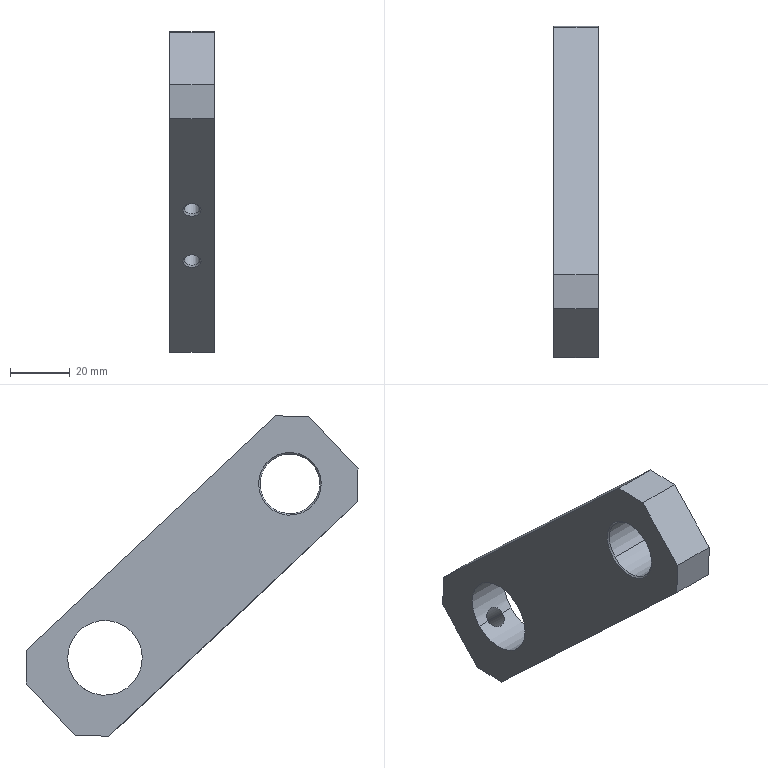Component | SolidWorks | FilmMechanism-3-1_LeftSupportBlock-1 | 1 solid | 32 faces | box 15 x 111.11 x 107.26 mm | volume 62724 mm3 | cone 12 | cylinder 10 | plane 10 | commonest cylinder face diameters 5 x4 6.8 x2 25 x2 20 x2
STEP:
#1=COLOUR_RGB('',0.7922,0.8196,0.9333);
#2=FILL_AREA_STYLE_COLOUR('',#1);
#3=FILL_AREA_STYLE('',(#2));
#4=SURFACE_STYLE_FILL_AREA(#3);
#5=SURFACE_SIDE_STYLE('',(#4));
#6=SURFACE_STYLE_USAGE(.BOTH.,#5);
#7=PRESENTATION_STYLE_ASSIGNMENT((#6));
#8=CARTESIAN_POINT('',(-21.419,17.638,-2.001));
#9=VERTEX_POINT('',#8);
#10=CARTESIAN_POINT('',(-21.222,17.638,-2.001));
#11=VERTEX_POINT('',#10);
#12=CARTESIAN_POINT('',(-21.321,17.638,-2.001));
#13=DIRECTION('',(0.,-0.6854,-0.7282));
#14=DIRECTION('',(1.,0.,0.));
#15=AXIS2_PLACEMENT_3D('',#12,#13,#14);
#16=CIRCLE('',#15,0.09843);
#17=EDGE_CURVE('',#9,#11,#16,.T.);
#18=ORIENTED_EDGE('',*,*,#17,.F.);
#19=CARTESIAN_POINT('',(-21.44,17.624,-2.016));
#20=VERTEX_POINT('',#19);
#21=CARTESIAN_POINT('',(-21.44,17.624,-2.016));
#22=DIRECTION('',(-0.7071,-0.4846,-0.5149));
#23=VECTOR('',#22,39.37);
#24=LINE('',#21,#23);
#25=EDGE_CURVE('',#9,#20,#24,.T.);
#26=ORIENTED_EDGE('',*,*,#25,.T.);
#27=CARTESIAN_POINT('',(-21.202,17.624,-2.016));
#28=VERTEX_POINT('',#27);
#29=CARTESIAN_POINT('',(-21.321,17.624,-2.016));
#30=DIRECTION('',(0.,-0.6854,-0.7282));
#31=DIRECTION('',(1.,0.,0.));
#32=AXIS2_PLACEMENT_3D('',#29,#30,#31);
#33=CIRCLE('',#32,0.1191);
#34=EDGE_CURVE('',#20,#28,#33,.T.);
#35=ORIENTED_EDGE('',*,*,#34,.T.);
#36=CARTESIAN_POINT('',(-21.202,17.624,-2.016));
#37=DIRECTION('',(0.7071,-0.4846,-0.5149));
#38=VECTOR('',#37,39.37);
#39=LINE('',#36,#38);
#40=EDGE_CURVE('',#11,#28,#39,.T.);
#41=ORIENTED_EDGE('',*,*,#40,.F.);
#42=EDGE_LOOP('',(#18,#26,#35,#41));
#43=FACE_OUTER_BOUND('',#42,.T.);
#44=CARTESIAN_POINT('',(-21.321,17.624,-2.016));
#45=DIRECTION('',(0.,-0.6854,-0.7282));
#46=DIRECTION('',(1.,0.,0.));
#47=AXIS2_PLACEMENT_3D('',#44,#45,#46);
#48=CONICAL_SURFACE('',#47,0.1191,0.7854);
#49=ADVANCED_FACE('',(#43),#48,.F.);
#50=CARTESIAN_POINT('',(-21.419,18.163,-1.443));
#51=VERTEX_POINT('',#50);
#52=CARTESIAN_POINT('',(-21.222,18.163,-1.443));
#53=VERTEX_POINT('',#52);
#54=CARTESIAN_POINT('',(-21.321,18.163,-1.443));
#55=DIRECTION('',(0.,-0.6854,-0.7282));
#56=DIRECTION('',(1.,0.,0.));
#57=AXIS2_PLACEMENT_3D('',#54,#55,#56);
#58=CIRCLE('',#57,0.09843);
#59=EDGE_CURVE('',#51,#53,#58,.T.);
#60=ORIENTED_EDGE('',*,*,#59,.F.);
#61=CARTESIAN_POINT('',(-21.419,17.624,-2.016));
#62=DIRECTION('',(0.,-0.6854,-0.7282));
#63=VECTOR('',#62,39.37);
#64=LINE('',#61,#63);
#65=EDGE_CURVE('',#51,#9,#64,.T.);
#66=ORIENTED_EDGE('',*,*,#65,.T.);
#67=ORIENTED_EDGE('',*,*,#17,.T.);
#68=CARTESIAN_POINT('',(-21.222,17.624,-2.016));
#69=DIRECTION('',(0.,-0.6854,-0.7282));
#70=VECTOR('',#69,39.37);
#71=LINE('',#68,#70);
#72=EDGE_CURVE('',#53,#11,#71,.T.);
#73=ORIENTED_EDGE('',*,*,#72,.F.);
#74=EDGE_LOOP('',(#60,#66,#67,#73));
#75=FACE_OUTER_BOUND('',#74,.T.);
#76=CARTESIAN_POINT('',(-21.321,17.624,-2.016));
#77=DIRECTION('',(0.,-0.6854,-0.7282));
#78=DIRECTION('',(1.,0.,0.));
#79=AXIS2_PLACEMENT_3D('',#76,#77,#78);
#80=CYLINDRICAL_SURFACE('',#79,0.09843);
#81=ADVANCED_FACE('',(#75),#80,.F.);
#82=CARTESIAN_POINT('',(-21.321,18.204,-1.4));
#83=VERTEX_POINT('',#82);
#84=CARTESIAN_POINT('',(-21.222,18.163,-1.443));
#85=DIRECTION('',(0.8572,-0.353,-0.375));
#86=VECTOR('',#85,39.37);
#87=LINE('',#84,#86);
#88=EDGE_CURVE('',#83,#53,#87,.T.);
#89=ORIENTED_EDGE('',*,*,#88,.F.);
#90=CARTESIAN_POINT('',(-21.419,18.163,-1.443));
#91=DIRECTION('',(-0.8572,-0.353,-0.375));
#92=VECTOR('',#91,39.37);
#93=LINE('',#90,#92);
#94=EDGE_CURVE('',#83,#51,#93,.T.);
#95=ORIENTED_EDGE('',*,*,#94,.T.);
#96=ORIENTED_EDGE('',*,*,#59,.T.);
#97=EDGE_LOOP('',(#89,#95,#96));
#98=FACE_OUTER_BOUND('',#97,.T.);
#99=CARTESIAN_POINT('',(-21.321,18.163,-1.443));
#100=DIRECTION('',(0.,-0.6854,-0.7282));
#101=DIRECTION('',(1.,0.,0.));
#102=AXIS2_PLACEMENT_3D('',#99,#100,#101);
#103=CONICAL_SURFACE('',#102,0.09843,1.03);
#104=ADVANCED_FACE('',(#98),#103,.F.);
#105=CARTESIAN_POINT('',(-21.419,16.921,-1.327));
#106=VERTEX_POINT('',#105);
#107=CARTESIAN_POINT('',(-21.222,16.921,-1.327));
#108=VERTEX_POINT('',#107);
#109=CARTESIAN_POINT('',(-21.321,16.921,-1.327));
#110=DIRECTION('',(0.,-0.6854,-0.7282));
#111=DIRECTION('',(1.,0.,0.));
#112=AXIS2_PLACEMENT_3D('',#109,#110,#111);
#113=CIRCLE('',#112,0.09843);
#114=EDGE_CURVE('',#106,#108,#113,.T.);
#115=ORIENTED_EDGE('',*,*,#114,.F.);
#116=CARTESIAN_POINT('',(-21.44,16.907,-1.342));
#117=VERTEX_POINT('',#116);
#118=CARTESIAN_POINT('',(-21.44,16.907,-1.342));
#119=DIRECTION('',(-0.7071,-0.4846,-0.5149));
#120=VECTOR('',#119,39.37);
#121=LINE('',#118,#120);
#122=EDGE_CURVE('',#106,#117,#121,.T.);
#123=ORIENTED_EDGE('',*,*,#122,.T.);
#124=CARTESIAN_POINT('',(-21.202,16.907,-1.342));
#125=VERTEX_POINT('',#124);
#126=CARTESIAN_POINT('',(-21.321,16.907,-1.342));
#127=DIRECTION('',(0.,-0.6854,-0.7282));
#128=DIRECTION('',(1.,0.,0.));
#129=AXIS2_PLACEMENT_3D('',#126,#127,#128);
#130=CIRCLE('',#129,0.1191);
#131=EDGE_CURVE('',#117,#125,#130,.T.);
#132=ORIENTED_EDGE('',*,*,#131,.T.);
#133=CARTESIAN_POINT('',(-21.202,16.907,-1.342));
#134=DIRECTION('',(0.7071,-0.4846,-0.5149));
#135=VECTOR('',#134,39.37);
#136=LINE('',#133,#135);
#137=EDGE_CURVE('',#108,#125,#136,.T.);
#138=ORIENTED_EDGE('',*,*,#137,.F.);
#139=EDGE_LOOP('',(#115,#123,#132,#138));
#140=FACE_OUTER_BOUND('',#139,.T.);
#141=CARTESIAN_POINT('',(-21.321,16.907,-1.342));
#142=DIRECTION('',(0.,-0.6854,-0.7282));
#143=DIRECTION('',(1.,0.,0.));
#144=AXIS2_PLACEMENT_3D('',#141,#142,#143);
#145=CONICAL_SURFACE('',#144,0.1191,0.7854);
#146=ADVANCED_FACE('',(#140),#145,.F.);
#147=CARTESIAN_POINT('',(-21.419,17.447,-0.7684));
#148=VERTEX_POINT('',#147);
#149=CARTESIAN_POINT('',(-21.222,17.447,-0.7684));
#150=VERTEX_POINT('',#149);
#151=CARTESIAN_POINT('',(-21.321,17.447,-0.7684));
#152=DIRECTION('',(0.,-0.6854,-0.7282));
#153=DIRECTION('',(1.,0.,0.));
#154=AXIS2_PLACEMENT_3D('',#151,#152,#153);
#155=CIRCLE('',#154,0.09843);
#156=EDGE_CURVE('',#148,#150,#155,.T.);
#157=ORIENTED_EDGE('',*,*,#156,.F.);
#158=CARTESIAN_POINT('',(-21.419,16.907,-1.342));
#159=DIRECTION('',(0.,-0.6854,-0.7282));
#160=VECTOR('',#159,39.37);
#161=LINE('',#158,#160);
#162=EDGE_CURVE('',#148,#106,#161,.T.);
#163=ORIENTED_EDGE('',*,*,#162,.T.);
#164=ORIENTED_EDGE('',*,*,#114,.T.);
#165=CARTESIAN_POINT('',(-21.222,16.907,-1.342));
#166=DIRECTION('',(0.,-0.6854,-0.7282));
#167=VECTOR('',#166,39.37);
#168=LINE('',#165,#167);
#169=EDGE_CURVE('',#150,#108,#168,.T.);
#170=ORIENTED_EDGE('',*,*,#169,.F.);
#171=EDGE_LOOP('',(#157,#163,#164,#170));
#172=FACE_OUTER_BOUND('',#171,.T.);
#173=CARTESIAN_POINT('',(-21.321,16.907,-1.342));
#174=DIRECTION('',(0.,-0.6854,-0.7282));
#175=DIRECTION('',(1.,0.,0.));
#176=AXIS2_PLACEMENT_3D('',#173,#174,#175);
#177=CYLINDRICAL_SURFACE('',#176,0.09843);
#178=ADVANCED_FACE('',(#172),#177,.F.);
#179=CARTESIAN_POINT('',(-21.321,17.487,-0.7253));
#180=VERTEX_POINT('',#179);
#181=CARTESIAN_POINT('',(-21.222,17.447,-0.7684));
#182=DIRECTION('',(0.8572,-0.353,-0.375));
#183=VECTOR('',#182,39.37);
#184=LINE('',#181,#183);
#185=EDGE_CURVE('',#180,#150,#184,.T.);
#186=ORIENTED_EDGE('',*,*,#185,.F.);
#187=CARTESIAN_POINT('',(-21.419,17.447,-0.7684));
#188=DIRECTION('',(-0.8572,-0.353,-0.375));
#189=VECTOR('',#188,39.37);
#190=LINE('',#187,#189);
#191=EDGE_CURVE('',#180,#148,#190,.T.);
#192=ORIENTED_EDGE('',*,*,#191,.T.);
#193=ORIENTED_EDGE('',*,*,#156,.T.);
#194=EDGE_LOOP('',(#186,#192,#193));
#195=FACE_OUTER_BOUND('',#194,.T.);
#196=CARTESIAN_POINT('',(-21.321,17.447,-0.7684));
#197=DIRECTION('',(0.,-0.6854,-0.7282));
#198=DIRECTION('',(1.,0.,0.));
#199=AXIS2_PLACEMENT_3D('',#196,#197,#198);
#200=CONICAL_SURFACE('',#199,0.09843,1.03);
#201=ADVANCED_FACE('',(#195),#200,.F.);
#202=CARTESIAN_POINT('',(-21.187,19.651,-2.843));
#203=VERTEX_POINT('',#202);
#204=CARTESIAN_POINT('',(-21.455,19.651,-2.843));
#205=VERTEX_POINT('',#204);
#206=CARTESIAN_POINT('',(-21.321,19.651,-2.843));
#207=DIRECTION('',(-0.,0.7282,-0.6854));
#208=DIRECTION('',(-1.,0.,0.));
#209=AXIS2_PLACEMENT_3D('',#206,#207,#208);
#210=CIRCLE('',#209,0.1339);
#211=EDGE_CURVE('',#203,#205,#210,.T.);
#212=ORIENTED_EDGE('',*,*,#211,.F.);
#213=CARTESIAN_POINT('',(-21.162,19.668,-2.86));
#214=VERTEX_POINT('',#213);
#215=CARTESIAN_POINT('',(-21.162,19.668,-2.86));
#216=DIRECTION('',(0.7071,0.5149,-0.4846));
#217=VECTOR('',#216,39.37);
#218=LINE('',#215,#217);
#219=EDGE_CURVE('',#203,#214,#218,.T.);
#220=ORIENTED_EDGE('',*,*,#219,.T.);
#221=CARTESIAN_POINT('',(-21.479,19.668,-2.86));
#222=VERTEX_POINT('',#221);
#223=CARTESIAN_POINT('',(-21.321,19.668,-2.86));
#224=DIRECTION('',(-0.,0.7282,-0.6854));
#225=DIRECTION('',(-1.,0.,0.));
#226=AXIS2_PLACEMENT_3D('',#223,#224,#225);
#227=CIRCLE('',#226,0.1585);
#228=EDGE_CURVE('',#214,#222,#227,.T.);
#229=ORIENTED_EDGE('',*,*,#228,.T.);
#230=CARTESIAN_POINT('',(-21.479,19.668,-2.86));
#231=DIRECTION('',(-0.7071,0.5149,-0.4846));
#232=VECTOR('',#231,39.37);
#233=LINE('',#230,#232);
#234=EDGE_CURVE('',#205,#222,#233,.T.);
#235=ORIENTED_EDGE('',*,*,#234,.F.);
#236=EDGE_LOOP('',(#212,#220,#229,#235));
#237=FACE_OUTER_BOUND('',#236,.T.);
#238=CARTESIAN_POINT('',(-21.321,19.668,-2.86));
#239=DIRECTION('',(-0.,0.7282,-0.6854));
#240=DIRECTION('',(-1.,0.,0.));
#241=AXIS2_PLACEMENT_3D('',#238,#239,#240);
#242=CONICAL_SURFACE('',#241,0.1585,0.7854);
#243=ADVANCED_FACE('',(#237),#242,.F.);
#244=CARTESIAN_POINT('',(-21.187,19.31,-2.522));
#245=VERTEX_POINT('',#244);
#246=CARTESIAN_POINT('',(-21.455,19.31,-2.522));
#247=VERTEX_POINT('',#246);
#248=CARTESIAN_POINT('',(-21.187,19.31,-2.522));
#249=CARTESIAN_POINT('',(-21.187,19.304,-2.529));
#250=CARTESIAN_POINT('',(-21.188,19.298,-2.535));
#251=CARTESIAN_POINT('',(-21.191,19.285,-2.547));
#252=CARTESIAN_POINT('',(-21.194,19.279,-2.553));
#253=CARTESIAN_POINT('',(-21.2,19.267,-2.563));
#254=CARTESIAN_POINT('',(-21.205,19.261,-2.568));
#255=CARTESIAN_POINT('',(-21.214,19.249,-2.577));
#256=CARTESIAN_POINT('',(-21.22,19.244,-2.581));
#257=CARTESIAN_POINT('',(-21.232,19.233,-2.589));
#258=CARTESIAN_POINT('',(-21.239,19.229,-2.592));
#259=CARTESIAN_POINT('',(-21.253,19.22,-2.597));
#260=CARTESIAN_POINT('',(-21.261,19.217,-2.6));
#261=CARTESIAN_POINT('',(-21.277,19.211,-2.603));
#262=CARTESIAN_POINT('',(-21.286,19.209,-2.605));
#263=CARTESIAN_POINT('',(-21.303,19.206,-2.607));
#264=CARTESIAN_POINT('',(-21.312,19.205,-2.607));
#265=CARTESIAN_POINT('',(-21.33,19.205,-2.607));
#266=CARTESIAN_POINT('',(-21.338,19.206,-2.607));
#267=CARTESIAN_POINT('',(-21.355,19.209,-2.605));
#268=CARTESIAN_POINT('',(-21.364,19.211,-2.603));
#269=CARTESIAN_POINT('',(-21.38,19.217,-2.6));
#270=CARTESIAN_POINT('',(-21.388,19.22,-2.597));
#271=CARTESIAN_POINT('',(-21.402,19.229,-2.592));
#272=CARTESIAN_POINT('',(-21.409,19.233,-2.589));
#273=CARTESIAN_POINT('',(-21.421,19.244,-2.581));
#274=CARTESIAN_POINT('',(-21.427,19.249,-2.577));
#275=CARTESIAN_POINT('',(-21.437,19.261,-2.568));
#276=CARTESIAN_POINT('',(-21.441,19.267,-2.563));
#277=CARTESIAN_POINT('',(-21.448,19.279,-2.553));
#278=CARTESIAN_POINT('',(-21.45,19.285,-2.547));
#279=CARTESIAN_POINT('',(-21.454,19.298,-2.535));
#280=CARTESIAN_POINT('',(-21.455,19.304,-2.529));
#281=CARTESIAN_POINT('',(-21.455,19.31,-2.522));
#282=B_SPLINE_CURVE_WITH_KNOTS('',3,(#248,#249,#250,#251,#252,#253,#254,#255,#256,#257,#258,#259,#260,#261,#262,#263,#264,#265,#266,#267,#268,#269,#270,#271,#272,#273,#274,#275,#276,#277,#278,#279,#280,#281),.UNSPECIFIED.,.F.,.F.,(4,2,2,2,2,2,2,2,2,2,2,2,2,2,2,2,4),(0.01068,0.01135,0.01202,0.01268,0.01335,0.01402,0.01468,0.01535,0.01602,0.01669,0.01735,0.01802,0.01869,0.01936,0.02002,0.02069,0.02136),.UNSPECIFIED.);
#283=EDGE_CURVE('',#245,#247,#282,.T.);
#284=ORIENTED_EDGE('',*,*,#283,.F.);
#285=CARTESIAN_POINT('',(-21.187,19.668,-2.86));
#286=DIRECTION('',(-0.,0.7282,-0.6854));
#287=VECTOR('',#286,39.37);
#288=LINE('',#285,#287);
#289=EDGE_CURVE('',#245,#203,#288,.T.);
#290=ORIENTED_EDGE('',*,*,#289,.T.);
#291=ORIENTED_EDGE('',*,*,#211,.T.);
#292=CARTESIAN_POINT('',(-21.455,19.668,-2.86));
#293=DIRECTION('',(-0.,0.7282,-0.6854));
#294=VECTOR('',#293,39.37);
#295=LINE('',#292,#294);
#296=EDGE_CURVE('',#247,#205,#295,.T.);
#297=ORIENTED_EDGE('',*,*,#296,.F.);
#298=EDGE_LOOP('',(#284,#290,#291,#297));
#299=FACE_OUTER_BOUND('',#298,.T.);
#300=CARTESIAN_POINT('',(-21.321,19.668,-2.86));
#301=DIRECTION('',(-0.,0.7282,-0.6854));
#302=DIRECTION('',(-1.,0.,0.));
#303=AXIS2_PLACEMENT_3D('',#300,#301,#302);
#304=CYLINDRICAL_SURFACE('',#303,0.1339);
#305=ADVANCED_FACE('',(#299),#304,.F.);
#306=CARTESIAN_POINT('',(-21.616,18.593,-1.848));
#307=VERTEX_POINT('',#306);
#308=CARTESIAN_POINT('',(-21.616,19.31,-2.522));
#309=VERTEX_POINT('',#308);
#310=CARTESIAN_POINT('',(-21.616,18.952,-2.185));
#311=DIRECTION('',(1.,0.,0.));
#312=DIRECTION('',(0.,0.7282,-0.6854));
#313=AXIS2_PLACEMENT_3D('',#310,#311,#312);
#314=CIRCLE('',#313,0.4921);
#315=EDGE_CURVE('',#307,#309,#314,.T.);
#316=ORIENTED_EDGE('',*,*,#315,.F.);
#317=CARTESIAN_POINT('',(-21.025,18.593,-1.848));
#318=VERTEX_POINT('',#317);
#319=CARTESIAN_POINT('',(-21.025,18.593,-1.848));
#320=DIRECTION('',(1.,0.,0.));
#321=VECTOR('',#320,39.37);
#322=LINE('',#319,#321);
#323=EDGE_CURVE('',#307,#318,#322,.T.);
#324=ORIENTED_EDGE('',*,*,#323,.T.);
#325=CARTESIAN_POINT('',(-21.025,19.31,-2.522));
#326=VERTEX_POINT('',#325);
#327=CARTESIAN_POINT('',(-21.025,18.952,-2.185));
#328=DIRECTION('',(1.,0.,0.));
#329=DIRECTION('',(0.,0.7282,-0.6854));
#330=AXIS2_PLACEMENT_3D('',#327,#328,#329);
#331=CIRCLE('',#330,0.4921);
#332=EDGE_CURVE('',#318,#326,#331,.T.);
#333=ORIENTED_EDGE('',*,*,#332,.T.);
#334=CARTESIAN_POINT('',(-21.025,19.31,-2.522));
#335=DIRECTION('',(1.,0.,0.));
#336=VECTOR('',#335,39.37);
#337=LINE('',#334,#336);
#338=EDGE_CURVE('',#245,#326,#337,.T.);
#339=ORIENTED_EDGE('',*,*,#338,.F.);
#340=ORIENTED_EDGE('',*,*,#283,.T.);
#341=CARTESIAN_POINT('',(-21.025,19.31,-2.522));
#342=DIRECTION('',(1.,0.,0.));
#343=VECTOR('',#342,39.37);
#344=LINE('',#341,#343);
#345=EDGE_CURVE('',#309,#247,#344,.T.);
#346=ORIENTED_EDGE('',*,*,#345,.F.);
#347=EDGE_LOOP('',(#316,#324,#333,#339,#340,#346));
#348=FACE_OUTER_BOUND('',#347,.T.);
#349=CARTESIAN_POINT('',(-21.025,18.952,-2.185));
#350=DIRECTION('',(1.,0.,0.));
#351=DIRECTION('',(0.,0.7282,-0.6854));
#352=AXIS2_PLACEMENT_3D('',#349,#350,#351);
#353=CYLINDRICAL_SURFACE('',#352,0.4921);
#354=ADVANCED_FACE('',(#348),#353,.F.);
#355=CARTESIAN_POINT('',(-21.596,16.802,-0.1613));
#356=VERTEX_POINT('',#355);
#357=CARTESIAN_POINT('',(-21.596,16.228,0.3784));
#358=VERTEX_POINT('',#357);
#359=CARTESIAN_POINT('',(-21.596,16.515,0.1086));
#360=DIRECTION('',(-1.,-0.,-0.));
#361=DIRECTION('',(0.,-0.7282,0.6854));
#362=AXIS2_PLACEMENT_3D('',#359,#360,#361);
#363=CIRCLE('',#362,0.3937);
#364=EDGE_CURVE('',#356,#358,#363,.T.);
#365=ORIENTED_EDGE('',*,*,#364,.F.);
#366=CARTESIAN_POINT('',(-21.616,16.816,-0.1748));
#367=VERTEX_POINT('',#366);
#368=CARTESIAN_POINT('',(-21.616,16.816,-0.1748));
#369=DIRECTION('',(-0.7071,0.5149,-0.4846));
#370=VECTOR('',#369,39.37);
#371=LINE('',#368,#370);
#372=EDGE_CURVE('',#356,#367,#371,.T.);
#373=ORIENTED_EDGE('',*,*,#372,.T.);
#374=CARTESIAN_POINT('',(-21.616,16.214,0.3919));
#375=VERTEX_POINT('',#374);
#376=CARTESIAN_POINT('',(-21.616,16.515,0.1086));
#377=DIRECTION('',(-1.,-0.,-0.));
#378=DIRECTION('',(0.,-0.7282,0.6854));
#379=AXIS2_PLACEMENT_3D('',#376,#377,#378);
#380=CIRCLE('',#379,0.4134);
#381=EDGE_CURVE('',#367,#375,#380,.T.);
#382=ORIENTED_EDGE('',*,*,#381,.T.);
#383=CARTESIAN_POINT('',(-21.616,16.214,0.3919));
#384=DIRECTION('',(-0.7071,-0.5149,0.4846));
#385=VECTOR('',#384,39.37);
#386=LINE('',#383,#385);
#387=EDGE_CURVE('',#358,#375,#386,.T.);
#388=ORIENTED_EDGE('',*,*,#387,.F.);
#389=EDGE_LOOP('',(#365,#373,#382,#388));
#390=FACE_OUTER_BOUND('',#389,.T.);
#391=CARTESIAN_POINT('',(-21.616,16.515,0.1086));
#392=DIRECTION('',(-1.,-0.,-0.));
#393=DIRECTION('',(0.,-0.7282,0.6854));
#394=AXIS2_PLACEMENT_3D('',#391,#392,#393);
#395=CONICAL_SURFACE('',#394,0.4134,0.7854);
#396=ADVANCED_FACE('',(#390),#395,.F.);
#397=CARTESIAN_POINT('',(-21.025,16.802,-0.1613));
#398=VERTEX_POINT('',#397);
#399=CARTESIAN_POINT('',(-21.025,16.228,0.3784));
#400=VERTEX_POINT('',#399);
#401=CARTESIAN_POINT('',(-21.025,16.515,0.1086));
#402=DIRECTION('',(-1.,-0.,-0.));
#403=DIRECTION('',(0.,-0.7282,0.6854));
#404=AXIS2_PLACEMENT_3D('',#401,#402,#403);
#405=CIRCLE('',#404,0.3937);
#406=EDGE_CURVE('',#398,#400,#405,.T.);
#407=ORIENTED_EDGE('',*,*,#406,.F.);
#408=CARTESIAN_POINT('',(-21.616,16.802,-0.1613));
#409=DIRECTION('',(-1.,-0.,-0.));
#410=VECTOR('',#409,39.37);
#411=LINE('',#408,#410);
#412=EDGE_CURVE('',#398,#356,#411,.T.);
#413=ORIENTED_EDGE('',*,*,#412,.T.);
#414=ORIENTED_EDGE('',*,*,#364,.T.);
#415=CARTESIAN_POINT('',(-21.616,16.228,0.3784));
#416=DIRECTION('',(-1.,-0.,-0.));
#417=VECTOR('',#416,39.37);
#418=LINE('',#415,#417);
#419=EDGE_CURVE('',#400,#358,#418,.T.);
#420=ORIENTED_EDGE('',*,*,#419,.F.);
#421=EDGE_LOOP('',(#407,#413,#414,#420));
#422=FACE_OUTER_BOUND('',#421,.T.);
#423=CARTESIAN_POINT('',(-21.616,16.515,0.1086));
#424=DIRECTION('',(-1.,-0.,-0.));
#425=DIRECTION('',(0.,-0.7282,0.6854));
#426=AXIS2_PLACEMENT_3D('',#423,#424,#425);
#427=CYLINDRICAL_SURFACE('',#426,0.3937);
#428=ADVANCED_FACE('',(#422),#427,.F.);
#429=CARTESIAN_POINT('',(-21.616,19.979,-2.07));
#430=VERTEX_POINT('',#429);
#431=CARTESIAN_POINT('',(-21.616,19.992,-2.516));
#432=VERTEX_POINT('',#431);
#433=CARTESIAN_POINT('',(-21.616,19.979,-2.07));
#434=DIRECTION('',(-0.,0.03026,-0.9995));
#435=VECTOR('',#434,39.37);
#436=LINE('',#433,#435);
#437=EDGE_CURVE('',#430,#432,#436,.T.);
#438=ORIENTED_EDGE('',*,*,#437,.F.);
#439=CARTESIAN_POINT('',(-21.025,19.979,-2.07));
#440=VERTEX_POINT('',#439);
#441=CARTESIAN_POINT('',(-21.025,19.979,-2.07));
#442=DIRECTION('',(-1.,-0.,-0.));
#443=VECTOR('',#442,39.37);
#444=LINE('',#441,#443);
#445=EDGE_CURVE('',#440,#430,#444,.T.);
#446=ORIENTED_EDGE('',*,*,#445,.F.);
#447=CARTESIAN_POINT('',(-21.025,19.992,-2.516));
#448=VERTEX_POINT('',#447);
#449=CARTESIAN_POINT('',(-21.025,19.979,-2.07));
#450=DIRECTION('',(-0.,0.03026,-0.9995));
#451=VECTOR('',#450,39.37);
#452=LINE('',#449,#451);
#453=EDGE_CURVE('',#440,#448,#452,.T.);
#454=ORIENTED_EDGE('',*,*,#453,.T.);
#455=CARTESIAN_POINT('',(-21.025,19.992,-2.516));
#456=DIRECTION('',(-1.,-0.,-0.));
#457=VECTOR('',#456,39.37);
#458=LINE('',#455,#457);
#459=EDGE_CURVE('',#448,#432,#458,.T.);
#460=ORIENTED_EDGE('',*,*,#459,.T.);
#461=EDGE_LOOP('',(#438,#446,#454,#460));
#462=FACE_OUTER_BOUND('',#461,.T.);
#463=CARTESIAN_POINT('',(-21.025,19.979,-2.07));
#464=DIRECTION('',(-0.,0.9995,0.03026));
#465=DIRECTION('',(-0.,0.03026,-0.9995));
#466=AXIS2_PLACEMENT_3D('',#463,#464,#465);
#467=PLANE('',#466);
#468=ADVANCED_FACE('',(#462),#467,.T.);
#469=CARTESIAN_POINT('',(-21.616,16.711,1.006));
#470=VERTEX_POINT('',#469);
#471=CARTESIAN_POINT('',(-21.616,16.711,1.006));
#472=DIRECTION('',(-0.,0.7282,-0.6854));
#473=VECTOR('',#472,39.37);
#474=LINE('',#471,#473);
#475=EDGE_CURVE('',#470,#430,#474,.T.);
#476=ORIENTED_EDGE('',*,*,#475,.F.);
#477=CARTESIAN_POINT('',(-21.025,16.711,1.006));
#478=VERTEX_POINT('',#477);
#479=CARTESIAN_POINT('',(-21.025,16.711,1.006));
#480=DIRECTION('',(-1.,-0.,-0.));
#481=VECTOR('',#480,39.37);
#482=LINE('',#479,#481);
#483=EDGE_CURVE('',#478,#470,#482,.T.);
#484=ORIENTED_EDGE('',*,*,#483,.F.);
#485=CARTESIAN_POINT('',(-21.025,16.711,1.006));
#486=DIRECTION('',(-0.,0.7282,-0.6854));
#487=VECTOR('',#486,39.37);
#488=LINE('',#485,#487);
#489=EDGE_CURVE('',#478,#440,#488,.T.);
#490=ORIENTED_EDGE('',*,*,#489,.T.);
#491=ORIENTED_EDGE('',*,*,#445,.T.);
#492=EDGE_LOOP('',(#476,#484,#490,#491));
#493=FACE_OUTER_BOUND('',#492,.T.);
#494=CARTESIAN_POINT('',(-21.025,16.711,1.006));
#495=DIRECTION('',(-0.,0.6854,0.7282));
#496=DIRECTION('',(-1.,-0.,-0.));
#497=AXIS2_PLACEMENT_3D('',#494,#495,#496);
#498=PLANE('',#497);
#499=ADVANCED_FACE('',(#493),#498,.T.);
#500=CARTESIAN_POINT('',(-21.616,16.265,0.9923));
#501=VERTEX_POINT('',#500);
#502=CARTESIAN_POINT('',(-21.616,16.265,0.9923));
#503=DIRECTION('',(-0.,0.9995,0.03026));
#504=VECTOR('',#503,39.37);
#505=LINE('',#502,#504);
#506=EDGE_CURVE('',#501,#470,#505,.T.);
#507=ORIENTED_EDGE('',*,*,#506,.F.);
#508=CARTESIAN_POINT('',(-21.025,16.265,0.9923));
#509=VERTEX_POINT('',#508);
#510=CARTESIAN_POINT('',(-21.025,16.265,0.9923));
#511=DIRECTION('',(-1.,-0.,-0.));
#512=VECTOR('',#511,39.37);
#513=LINE('',#510,#512);
#514=EDGE_CURVE('',#509,#501,#513,.T.);
#515=ORIENTED_EDGE('',*,*,#514,.F.);
#516=CARTESIAN_POINT('',(-21.025,16.265,0.9923));
#517=DIRECTION('',(-0.,0.9995,0.03026));
#518=VECTOR('',#517,39.37);
#519=LINE('',#516,#518);
#520=EDGE_CURVE('',#509,#478,#519,.T.);
#521=ORIENTED_EDGE('',*,*,#520,.T.);
#522=ORIENTED_EDGE('',*,*,#483,.T.);
#523=EDGE_LOOP('',(#507,#515,#521,#522));
#524=FACE_OUTER_BOUND('',#523,.T.);
#525=CARTESIAN_POINT('',(-21.025,16.265,0.9923));
#526=DIRECTION('',(0.,-0.03026,0.9995));
#527=DIRECTION('',(-0.,0.9995,0.03026));
#528=AXIS2_PLACEMENT_3D('',#525,#526,#527);
#529=PLANE('',#528);
#530=ADVANCED_FACE('',(#524),#529,.T.);
#531=CARTESIAN_POINT('',(-21.616,15.618,0.3042));
#532=VERTEX_POINT('',#531);
#533=CARTESIAN_POINT('',(-21.616,15.618,0.3042));
#534=DIRECTION('',(-0.,0.6854,0.7282));
#535=VECTOR('',#534,39.37);
#536=LINE('',#533,#535);
#537=EDGE_CURVE('',#532,#501,#536,.T.);
#538=ORIENTED_EDGE('',*,*,#537,.F.);
#539=CARTESIAN_POINT('',(-21.025,15.618,0.3042));
#540=VERTEX_POINT('',#539);
#541=CARTESIAN_POINT('',(-21.025,15.618,0.3042));
#542=DIRECTION('',(-1.,-0.,-0.));
#543=VECTOR('',#542,39.37);
#544=LINE('',#541,#543);
#545=EDGE_CURVE('',#540,#532,#544,.T.);
#546=ORIENTED_EDGE('',*,*,#545,.F.);
#547=CARTESIAN_POINT('',(-21.025,15.618,0.3042));
#548=DIRECTION('',(-0.,0.6854,0.7282));
#549=VECTOR('',#548,39.37);
#550=LINE('',#547,#549);
#551=EDGE_CURVE('',#540,#509,#550,.T.);
#552=ORIENTED_EDGE('',*,*,#551,.T.);
#553=ORIENTED_EDGE('',*,*,#514,.T.);
#554=EDGE_LOOP('',(#538,#546,#552,#553));
#555=FACE_OUTER_BOUND('',#554,.T.);
#556=CARTESIAN_POINT('',(-21.025,15.618,0.3042));
#557=DIRECTION('',(0.,-0.7282,0.6854));
#558=DIRECTION('',(1.,0.,0.));
#559=AXIS2_PLACEMENT_3D('',#556,#557,#558);
#560=PLANE('',#559);
#561=ADVANCED_FACE('',(#555),#560,.T.);
#562=CARTESIAN_POINT('',(-21.616,15.631,-0.141));
#563=VERTEX_POINT('',#562);
#564=CARTESIAN_POINT('',(-21.616,15.631,-0.141));
#565=DIRECTION('',(0.,-0.03026,0.9995));
#566=VECTOR('',#565,39.37);
#567=LINE('',#564,#566);
#568=EDGE_CURVE('',#563,#532,#567,.T.);
#569=ORIENTED_EDGE('',*,*,#568,.F.);
#570=CARTESIAN_POINT('',(-21.025,15.631,-0.141));
#571=VERTEX_POINT('',#570);
#572=CARTESIAN_POINT('',(-21.025,15.631,-0.141));
#573=DIRECTION('',(-1.,-0.,-0.));
#574=VECTOR('',#573,39.37);
#575=LINE('',#572,#574);
#576=EDGE_CURVE('',#571,#563,#575,.T.);
#577=ORIENTED_EDGE('',*,*,#576,.F.);
#578=CARTESIAN_POINT('',(-21.025,15.631,-0.141));
#579=DIRECTION('',(0.,-0.03026,0.9995));
#580=VECTOR('',#579,39.37);
#581=LINE('',#578,#580);
#582=EDGE_CURVE('',#571,#540,#581,.T.);
#583=ORIENTED_EDGE('',*,*,#582,.T.);
#584=ORIENTED_EDGE('',*,*,#545,.T.);
#585=EDGE_LOOP('',(#569,#577,#583,#584));
#586=FACE_OUTER_BOUND('',#585,.T.);
#587=CARTESIAN_POINT('',(-21.025,15.631,-0.141));
#588=DIRECTION('',(0.,-0.9995,-0.03026));
#589=DIRECTION('',(0.,-0.03026,0.9995));
#590=AXIS2_PLACEMENT_3D('',#587,#588,#589);
#591=PLANE('',#590);
#592=ADVANCED_FACE('',(#586),#591,.T.);
#593=CARTESIAN_POINT('',(-21.321,17.624,-2.016));
#594=DIRECTION('',(0.,-0.6854,-0.7282));
#595=DIRECTION('',(1.,0.,0.));
#596=AXIS2_PLACEMENT_3D('',#593,#594,#595);
#597=CIRCLE('',#596,0.1191);
#598=EDGE_CURVE('',#28,#20,#597,.T.);
#599=ORIENTED_EDGE('',*,*,#598,.F.);
#600=ORIENTED_EDGE('',*,*,#34,.F.);
#601=EDGE_LOOP('',(#599,#600));
#602=FACE_BOUND('',#601,.T.);
#603=CARTESIAN_POINT('',(-21.321,16.907,-1.342));
#604=DIRECTION('',(0.,-0.6854,-0.7282));
#605=DIRECTION('',(1.,0.,0.));
#606=AXIS2_PLACEMENT_3D('',#603,#604,#605);
#607=CIRCLE('',#606,0.1191);
#608=EDGE_CURVE('',#125,#117,#607,.T.);
#609=ORIENTED_EDGE('',*,*,#608,.F.);
#610=ORIENTED_EDGE('',*,*,#131,.F.);
#611=EDGE_LOOP('',(#609,#610));
#612=FACE_BOUND('',#611,.T.);
#613=CARTESIAN_POINT('',(-21.616,18.899,-3.217));
#614=VERTEX_POINT('',#613);
#615=CARTESIAN_POINT('',(-21.616,18.899,-3.217));
#616=DIRECTION('',(0.,-0.7282,0.6854));
#617=VECTOR('',#616,39.37);
#618=LINE('',#615,#617);
#619=EDGE_CURVE('',#614,#563,#618,.T.);
#620=ORIENTED_EDGE('',*,*,#619,.F.);
#621=CARTESIAN_POINT('',(-21.025,18.899,-3.217));
#622=VERTEX_POINT('',#621);
#623=CARTESIAN_POINT('',(-21.025,18.899,-3.217));
#624=DIRECTION('',(-1.,-0.,-0.));
#625=VECTOR('',#624,39.37);
#626=LINE('',#623,#625);
#627=EDGE_CURVE('',#622,#614,#626,.T.);
#628=ORIENTED_EDGE('',*,*,#627,.F.);
#629=CARTESIAN_POINT('',(-21.025,18.899,-3.217));
#630=DIRECTION('',(0.,-0.7282,0.6854));
#631=VECTOR('',#630,39.37);
#632=LINE('',#629,#631);
#633=EDGE_CURVE('',#622,#571,#632,.T.);
#634=ORIENTED_EDGE('',*,*,#633,.T.);
#635=ORIENTED_EDGE('',*,*,#576,.T.);
#636=EDGE_LOOP('',(#620,#628,#634,#635));
#637=FACE_OUTER_BOUND('',#636,.T.);
#638=CARTESIAN_POINT('',(-21.025,18.899,-3.217));
#639=DIRECTION('',(0.,-0.6854,-0.7282));
#640=DIRECTION('',(0.,-0.7282,0.6854));
#641=AXIS2_PLACEMENT_3D('',#638,#639,#640);
#642=PLANE('',#641);
#643=ADVANCED_FACE('',(#602,#612,#637),#642,.T.);
#644=CARTESIAN_POINT('',(-21.616,19.345,-3.204));
#645=VERTEX_POINT('',#644);
#646=CARTESIAN_POINT('',(-21.616,19.345,-3.204));
#647=DIRECTION('',(0.,-0.9995,-0.03026));
#648=VECTOR('',#647,39.37);
#649=LINE('',#646,#648);
#650=EDGE_CURVE('',#645,#614,#649,.T.);
#651=ORIENTED_EDGE('',*,*,#650,.F.);
#652=CARTESIAN_POINT('',(-21.025,19.345,-3.204));
#653=VERTEX_POINT('',#652);
#654=CARTESIAN_POINT('',(-21.025,19.345,-3.204));
#655=DIRECTION('',(-1.,-0.,-0.));
#656=VECTOR('',#655,39.37);
#657=LINE('',#654,#656);
#658=EDGE_CURVE('',#653,#645,#657,.T.);
#659=ORIENTED_EDGE('',*,*,#658,.F.);
#660=CARTESIAN_POINT('',(-21.025,19.345,-3.204));
#661=DIRECTION('',(0.,-0.9995,-0.03026));
#662=VECTOR('',#661,39.37);
#663=LINE('',#660,#662);
#664=EDGE_CURVE('',#653,#622,#663,.T.);
#665=ORIENTED_EDGE('',*,*,#664,.T.);
#666=ORIENTED_EDGE('',*,*,#627,.T.);
#667=EDGE_LOOP('',(#651,#659,#665,#666));
#668=FACE_OUTER_BOUND('',#667,.T.);
#669=CARTESIAN_POINT('',(-21.025,19.345,-3.204));
#670=DIRECTION('',(-0.,0.03026,-0.9995));
#671=DIRECTION('',(0.,-0.9995,-0.03026));
#672=AXIS2_PLACEMENT_3D('',#669,#670,#671);
#673=PLANE('',#672);
#674=ADVANCED_FACE('',(#668),#673,.T.);
#675=CARTESIAN_POINT('',(-21.321,19.668,-2.86));
#676=DIRECTION('',(-0.,0.7282,-0.6854));
#677=DIRECTION('',(-1.,0.,0.));
#678=AXIS2_PLACEMENT_3D('',#675,#676,#677);
#679=CIRCLE('',#678,0.1585);
#680=EDGE_CURVE('',#222,#214,#679,.T.);
#681=ORIENTED_EDGE('',*,*,#680,.F.);
#682=ORIENTED_EDGE('',*,*,#228,.F.);
#683=EDGE_LOOP('',(#681,#682));
#684=FACE_BOUND('',#683,.T.);
#685=CARTESIAN_POINT('',(-21.616,19.992,-2.516));
#686=DIRECTION('',(0.,-0.6854,-0.7282));
#687=VECTOR('',#686,39.37);
#688=LINE('',#685,#687);
#689=EDGE_CURVE('',#432,#645,#688,.T.);
#690=ORIENTED_EDGE('',*,*,#689,.F.);
#691=ORIENTED_EDGE('',*,*,#459,.F.);
#692=CARTESIAN_POINT('',(-21.025,19.992,-2.516));
#693=DIRECTION('',(0.,-0.6854,-0.7282));
#694=VECTOR('',#693,39.37);
#695=LINE('',#692,#694);
#696=EDGE_CURVE('',#448,#653,#695,.T.);
#697=ORIENTED_EDGE('',*,*,#696,.T.);
#698=ORIENTED_EDGE('',*,*,#658,.T.);
#699=EDGE_LOOP('',(#690,#691,#697,#698));
#700=FACE_OUTER_BOUND('',#699,.T.);
#701=CARTESIAN_POINT('',(-21.025,19.992,-2.516));
#702=DIRECTION('',(-0.,0.7282,-0.6854));
#703=DIRECTION('',(-1.,-0.,-0.));
#704=AXIS2_PLACEMENT_3D('',#701,#702,#703);
#705=PLANE('',#704);
#706=ADVANCED_FACE('',(#684,#700),#705,.T.);
#707=CARTESIAN_POINT('',(-21.025,18.952,-2.185));
#708=DIRECTION('',(1.,0.,0.));
#709=DIRECTION('',(0.,0.7282,-0.6854));
#710=AXIS2_PLACEMENT_3D('',#707,#708,#709);
#711=CIRCLE('',#710,0.4921);
#712=EDGE_CURVE('',#326,#318,#711,.T.);
#713=ORIENTED_EDGE('',*,*,#712,.F.);
#714=ORIENTED_EDGE('',*,*,#332,.F.);
#715=EDGE_LOOP('',(#713,#714));
#716=FACE_BOUND('',#715,.T.);
#717=CARTESIAN_POINT('',(-21.025,16.515,0.1086));
#718=DIRECTION('',(-1.,-0.,-0.));
#719=DIRECTION('',(0.,-0.7282,0.6854));
#720=AXIS2_PLACEMENT_3D('',#717,#718,#719);
#721=CIRCLE('',#720,0.3937);
#722=EDGE_CURVE('',#400,#398,#721,.T.);
#723=ORIENTED_EDGE('',*,*,#722,.T.);
#724=ORIENTED_EDGE('',*,*,#406,.T.);
#725=EDGE_LOOP('',(#723,#724));
#726=FACE_BOUND('',#725,.T.);
#727=ORIENTED_EDGE('',*,*,#453,.F.);
#728=ORIENTED_EDGE('',*,*,#489,.F.);
#729=ORIENTED_EDGE('',*,*,#520,.F.);
#730=ORIENTED_EDGE('',*,*,#551,.F.);
#731=ORIENTED_EDGE('',*,*,#582,.F.);
#732=ORIENTED_EDGE('',*,*,#633,.F.);
#733=ORIENTED_EDGE('',*,*,#664,.F.);
#734=ORIENTED_EDGE('',*,*,#696,.F.);
#735=EDGE_LOOP('',(#727,#728,#729,#730,#731,#732,#733,#734));
#736=FACE_OUTER_BOUND('',#735,.T.);
#737=CARTESIAN_POINT('',(-21.025,17.805,-1.106));
#738=DIRECTION('',(-1.,-0.,-0.));
#739=DIRECTION('',(0.,-0.7282,0.6854));
#740=AXIS2_PLACEMENT_3D('',#737,#738,#739);
#741=PLANE('',#740);
#742=ADVANCED_FACE('',(#716,#726,#736),#741,.F.);
#743=CARTESIAN_POINT('',(-21.616,18.952,-2.185));
#744=DIRECTION('',(1.,0.,0.));
#745=DIRECTION('',(0.,0.7282,-0.6854));
#746=AXIS2_PLACEMENT_3D('',#743,#744,#745);
#747=CIRCLE('',#746,0.4921);
#748=EDGE_CURVE('',#309,#307,#747,.T.);
#749=ORIENTED_EDGE('',*,*,#748,.T.);
#750=ORIENTED_EDGE('',*,*,#315,.T.);
#751=EDGE_LOOP('',(#749,#750));
#752=FACE_BOUND('',#751,.T.);
#753=CARTESIAN_POINT('',(-21.616,16.515,0.1086));
#754=DIRECTION('',(-1.,-0.,-0.));
#755=DIRECTION('',(0.,-0.7282,0.6854));
#756=AXIS2_PLACEMENT_3D('',#753,#754,#755);
#757=CIRCLE('',#756,0.4134);
#758=EDGE_CURVE('',#375,#367,#757,.T.);
#759=ORIENTED_EDGE('',*,*,#758,.F.);
#760=ORIENTED_EDGE('',*,*,#381,.F.);
#761=EDGE_LOOP('',(#759,#760));
#762=FACE_BOUND('',#761,.T.);
#763=ORIENTED_EDGE('',*,*,#437,.T.);
#764=ORIENTED_EDGE('',*,*,#689,.T.);
#765=ORIENTED_EDGE('',*,*,#650,.T.);
#766=ORIENTED_EDGE('',*,*,#619,.T.);
#767=ORIENTED_EDGE('',*,*,#568,.T.);
#768=ORIENTED_EDGE('',*,*,#537,.T.);
#769=ORIENTED_EDGE('',*,*,#506,.T.);
#770=ORIENTED_EDGE('',*,*,#475,.T.);
#771=EDGE_LOOP('',(#763,#764,#765,#766,#767,#768,#769,#770));
#772=FACE_OUTER_BOUND('',#771,.T.);
#773=CARTESIAN_POINT('',(-21.616,17.805,-1.106));
#774=DIRECTION('',(-1.,-0.,-0.));
#775=DIRECTION('',(0.,-0.7282,0.6854));
#776=AXIS2_PLACEMENT_3D('',#773,#774,#775);
#777=PLANE('',#776);
#778=ADVANCED_FACE('',(#752,#762,#772),#777,.T.);
#779=ORIENTED_EDGE('',*,*,#412,.F.);
#780=ORIENTED_EDGE('',*,*,#722,.F.);
#781=ORIENTED_EDGE('',*,*,#419,.T.);
#782=CARTESIAN_POINT('',(-21.596,16.515,0.1086));
#783=DIRECTION('',(-1.,-0.,-0.));
#784=DIRECTION('',(0.,-0.7282,0.6854));
#785=AXIS2_PLACEMENT_3D('',#782,#783,#784);
#786=CIRCLE('',#785,0.3937);
#787=EDGE_CURVE('',#358,#356,#786,.T.);
#788=ORIENTED_EDGE('',*,*,#787,.T.);
#789=EDGE_LOOP('',(#779,#780,#781,#788));
#790=FACE_OUTER_BOUND('',#789,.T.);
#791=CARTESIAN_POINT('',(-21.616,16.515,0.1086));
#792=DIRECTION('',(-1.,-0.,-0.));
#793=DIRECTION('',(0.,-0.7282,0.6854));
#794=AXIS2_PLACEMENT_3D('',#791,#792,#793);
#795=CYLINDRICAL_SURFACE('',#794,0.3937);
#796=ADVANCED_FACE('',(#790),#795,.F.);
#797=ORIENTED_EDGE('',*,*,#372,.F.);
#798=ORIENTED_EDGE('',*,*,#787,.F.);
#799=ORIENTED_EDGE('',*,*,#387,.T.);
#800=ORIENTED_EDGE('',*,*,#758,.T.);
#801=EDGE_LOOP('',(#797,#798,#799,#800));
#802=FACE_OUTER_BOUND('',#801,.T.);
#803=CARTESIAN_POINT('',(-21.616,16.515,0.1086));
#804=DIRECTION('',(-1.,-0.,-0.));
#805=DIRECTION('',(0.,-0.7282,0.6854));
#806=AXIS2_PLACEMENT_3D('',#803,#804,#805);
#807=CONICAL_SURFACE('',#806,0.4134,0.7854);
#808=ADVANCED_FACE('',(#802),#807,.F.);
#809=ORIENTED_EDGE('',*,*,#323,.F.);
#810=ORIENTED_EDGE('',*,*,#748,.F.);
#811=ORIENTED_EDGE('',*,*,#345,.T.);
#812=CARTESIAN_POINT('',(-21.455,19.31,-2.522));
#813=CARTESIAN_POINT('',(-21.455,19.316,-2.516));
#814=CARTESIAN_POINT('',(-21.454,19.322,-2.509));
#815=CARTESIAN_POINT('',(-21.45,19.333,-2.496));
#816=CARTESIAN_POINT('',(-21.448,19.338,-2.49));
#817=CARTESIAN_POINT('',(-21.441,19.348,-2.477));
#818=CARTESIAN_POINT('',(-21.437,19.353,-2.47));
#819=CARTESIAN_POINT('',(-21.427,19.361,-2.458));
#820=CARTESIAN_POINT('',(-21.421,19.365,-2.452));
#821=CARTESIAN_POINT('',(-21.409,19.372,-2.442));
#822=CARTESIAN_POINT('',(-21.402,19.375,-2.437));
#823=CARTESIAN_POINT('',(-21.388,19.38,-2.428));
#824=CARTESIAN_POINT('',(-21.38,19.382,-2.425));
#825=CARTESIAN_POINT('',(-21.364,19.385,-2.418));
#826=CARTESIAN_POINT('',(-21.356,19.386,-2.416));
#827=CARTESIAN_POINT('',(-21.338,19.388,-2.413));
#828=CARTESIAN_POINT('',(-21.33,19.388,-2.412));
#829=CARTESIAN_POINT('',(-21.312,19.388,-2.412));
#830=CARTESIAN_POINT('',(-21.303,19.388,-2.413));
#831=CARTESIAN_POINT('',(-21.286,19.386,-2.416));
#832=CARTESIAN_POINT('',(-21.278,19.385,-2.418));
#833=CARTESIAN_POINT('',(-21.253,19.38,-2.428));
#834=CARTESIAN_POINT('',(-21.238,19.375,-2.436));
#835=CARTESIAN_POINT('',(-21.22,19.365,-2.452));
#836=CARTESIAN_POINT('',(-21.214,19.361,-2.458));
#837=CARTESIAN_POINT('',(-21.205,19.353,-2.47));
#838=CARTESIAN_POINT('',(-21.2,19.348,-2.477));
#839=CARTESIAN_POINT('',(-21.194,19.338,-2.49));
#840=CARTESIAN_POINT('',(-21.191,19.333,-2.496));
#841=CARTESIAN_POINT('',(-21.188,19.322,-2.509));
#842=CARTESIAN_POINT('',(-21.187,19.316,-2.516));
#843=CARTESIAN_POINT('',(-21.187,19.31,-2.522));
#844=B_SPLINE_CURVE_WITH_KNOTS('',3,(#812,#813,#814,#815,#816,#817,#818,#819,#820,#821,#822,#823,#824,#825,#826,#827,#828,#829,#830,#831,#832,#833,#834,#835,#836,#837,#838,#839,#840,#841,#842,#843),.UNSPECIFIED.,.F.,.F.,(4,2,2,2,2,2,2,2,2,2,2,2,2,2,2,4),(0.,0.0006675,0.001335,0.002003,0.00267,0.003338,0.004005,0.004673,0.00534,0.006008,0.006675,0.00801,0.008678,0.009345,0.01001,0.01068),.UNSPECIFIED.);
#845=EDGE_CURVE('',#247,#245,#844,.T.);
#846=ORIENTED_EDGE('',*,*,#845,.T.);
#847=ORIENTED_EDGE('',*,*,#338,.T.);
#848=ORIENTED_EDGE('',*,*,#712,.T.);
#849=EDGE_LOOP('',(#809,#810,#811,#846,#847,#848));
#850=FACE_OUTER_BOUND('',#849,.T.);
#851=CARTESIAN_POINT('',(-21.025,18.952,-2.185));
#852=DIRECTION('',(1.,0.,0.));
#853=DIRECTION('',(0.,0.7282,-0.6854));
#854=AXIS2_PLACEMENT_3D('',#851,#852,#853);
#855=CYLINDRICAL_SURFACE('',#854,0.4921);
#856=ADVANCED_FACE('',(#850),#855,.F.);
#857=ORIENTED_EDGE('',*,*,#289,.F.);
#858=ORIENTED_EDGE('',*,*,#845,.F.);
#859=ORIENTED_EDGE('',*,*,#296,.T.);
#860=CARTESIAN_POINT('',(-21.321,19.651,-2.843));
#861=DIRECTION('',(-0.,0.7282,-0.6854));
#862=DIRECTION('',(-1.,0.,0.));
#863=AXIS2_PLACEMENT_3D('',#860,#861,#862);
#864=CIRCLE('',#863,0.1339);
#865=EDGE_CURVE('',#205,#203,#864,.T.);
#866=ORIENTED_EDGE('',*,*,#865,.T.);
#867=EDGE_LOOP('',(#857,#858,#859,#866));
#868=FACE_OUTER_BOUND('',#867,.T.);
#869=CARTESIAN_POINT('',(-21.321,19.668,-2.86));
#870=DIRECTION('',(-0.,0.7282,-0.6854));
#871=DIRECTION('',(-1.,0.,0.));
#872=AXIS2_PLACEMENT_3D('',#869,#870,#871);
#873=CYLINDRICAL_SURFACE('',#872,0.1339);
#874=ADVANCED_FACE('',(#868),#873,.F.);
#875=ORIENTED_EDGE('',*,*,#219,.F.);
#876=ORIENTED_EDGE('',*,*,#865,.F.);
#877=ORIENTED_EDGE('',*,*,#234,.T.);
#878=ORIENTED_EDGE('',*,*,#680,.T.);
#879=EDGE_LOOP('',(#875,#876,#877,#878));
#880=FACE_OUTER_BOUND('',#879,.T.);
#881=CARTESIAN_POINT('',(-21.321,19.668,-2.86));
#882=DIRECTION('',(-0.,0.7282,-0.6854));
#883=DIRECTION('',(-1.,0.,0.));
#884=AXIS2_PLACEMENT_3D('',#881,#882,#883);
#885=CONICAL_SURFACE('',#884,0.1585,0.7854);
#886=ADVANCED_FACE('',(#880),#885,.F.);
#887=ORIENTED_EDGE('',*,*,#191,.F.);
#888=ORIENTED_EDGE('',*,*,#185,.T.);
#889=CARTESIAN_POINT('',(-21.321,17.447,-0.7684));
#890=DIRECTION('',(0.,-0.6854,-0.7282));
#891=DIRECTION('',(1.,0.,0.));
#892=AXIS2_PLACEMENT_3D('',#889,#890,#891);
#893=CIRCLE('',#892,0.09843);
#894=EDGE_CURVE('',#150,#148,#893,.T.);
#895=ORIENTED_EDGE('',*,*,#894,.T.);
#896=EDGE_LOOP('',(#887,#888,#895));
#897=FACE_OUTER_BOUND('',#896,.T.);
#898=CARTESIAN_POINT('',(-21.321,17.447,-0.7684));
#899=DIRECTION('',(0.,-0.6854,-0.7282));
#900=DIRECTION('',(1.,0.,0.));
#901=AXIS2_PLACEMENT_3D('',#898,#899,#900);
#902=CONICAL_SURFACE('',#901,0.09843,1.03);
#903=ADVANCED_FACE('',(#897),#902,.F.);
#904=ORIENTED_EDGE('',*,*,#162,.F.);
#905=ORIENTED_EDGE('',*,*,#894,.F.);
#906=ORIENTED_EDGE('',*,*,#169,.T.);
#907=CARTESIAN_POINT('',(-21.321,16.921,-1.327));
#908=DIRECTION('',(0.,-0.6854,-0.7282));
#909=DIRECTION('',(1.,0.,0.));
#910=AXIS2_PLACEMENT_3D('',#907,#908,#909);
#911=CIRCLE('',#910,0.09843);
#912=EDGE_CURVE('',#108,#106,#911,.T.);
#913=ORIENTED_EDGE('',*,*,#912,.T.);
#914=EDGE_LOOP('',(#904,#905,#906,#913));
#915=FACE_OUTER_BOUND('',#914,.T.);
#916=CARTESIAN_POINT('',(-21.321,16.907,-1.342));
#917=DIRECTION('',(0.,-0.6854,-0.7282));
#918=DIRECTION('',(1.,0.,0.));
#919=AXIS2_PLACEMENT_3D('',#916,#917,#918);
#920=CYLINDRICAL_SURFACE('',#919,0.09843);
#921=ADVANCED_FACE('',(#915),#920,.F.);
#922=ORIENTED_EDGE('',*,*,#122,.F.);
#923=ORIENTED_EDGE('',*,*,#912,.F.);
#924=ORIENTED_EDGE('',*,*,#137,.T.);
#925=ORIENTED_EDGE('',*,*,#608,.T.);
#926=EDGE_LOOP('',(#922,#923,#924,#925));
#927=FACE_OUTER_BOUND('',#926,.T.);
#928=CARTESIAN_POINT('',(-21.321,16.907,-1.342));
#929=DIRECTION('',(0.,-0.6854,-0.7282));
#930=DIRECTION('',(1.,0.,0.));
#931=AXIS2_PLACEMENT_3D('',#928,#929,#930);
#932=CONICAL_SURFACE('',#931,0.1191,0.7854);
#933=ADVANCED_FACE('',(#927),#932,.F.);
#934=ORIENTED_EDGE('',*,*,#94,.F.);
#935=ORIENTED_EDGE('',*,*,#88,.T.);
#936=CARTESIAN_POINT('',(-21.321,18.163,-1.443));
#937=DIRECTION('',(0.,-0.6854,-0.7282));
#938=DIRECTION('',(1.,0.,0.));
#939=AXIS2_PLACEMENT_3D('',#936,#937,#938);
#940=CIRCLE('',#939,0.09843);
#941=EDGE_CURVE('',#53,#51,#940,.T.);
#942=ORIENTED_EDGE('',*,*,#941,.T.);
#943=EDGE_LOOP('',(#934,#935,#942));
#944=FACE_OUTER_BOUND('',#943,.T.);
#945=CARTESIAN_POINT('',(-21.321,18.163,-1.443));
#946=DIRECTION('',(0.,-0.6854,-0.7282));
#947=DIRECTION('',(1.,0.,0.));
#948=AXIS2_PLACEMENT_3D('',#945,#946,#947);
#949=CONICAL_SURFACE('',#948,0.09843,1.03);
#950=ADVANCED_FACE('',(#944),#949,.F.);
#951=ORIENTED_EDGE('',*,*,#65,.F.);
#952=ORIENTED_EDGE('',*,*,#941,.F.);
#953=ORIENTED_EDGE('',*,*,#72,.T.);
#954=CARTESIAN_POINT('',(-21.321,17.638,-2.001));
#955=DIRECTION('',(0.,-0.6854,-0.7282));
#956=DIRECTION('',(1.,0.,0.));
#957=AXIS2_PLACEMENT_3D('',#954,#955,#956);
#958=CIRCLE('',#957,0.09843);
#959=EDGE_CURVE('',#11,#9,#958,.T.);
#960=ORIENTED_EDGE('',*,*,#959,.T.);
#961=EDGE_LOOP('',(#951,#952,#953,#960));
#962=FACE_OUTER_BOUND('',#961,.T.);
#963=CARTESIAN_POINT('',(-21.321,17.624,-2.016));
#964=DIRECTION('',(0.,-0.6854,-0.7282));
#965=DIRECTION('',(1.,0.,0.));
#966=AXIS2_PLACEMENT_3D('',#963,#964,#965);
#967=CYLINDRICAL_SURFACE('',#966,0.09843);
#968=ADVANCED_FACE('',(#962),#967,.F.);
#969=ORIENTED_EDGE('',*,*,#25,.F.);
#970=ORIENTED_EDGE('',*,*,#959,.F.);
#971=ORIENTED_EDGE('',*,*,#40,.T.);
#972=ORIENTED_EDGE('',*,*,#598,.T.);
#973=EDGE_LOOP('',(#969,#970,#971,#972));
#974=FACE_OUTER_BOUND('',#973,.T.);
#975=CARTESIAN_POINT('',(-21.321,17.624,-2.016));
#976=DIRECTION('',(0.,-0.6854,-0.7282));
#977=DIRECTION('',(1.,0.,0.));
#978=AXIS2_PLACEMENT_3D('',#975,#976,#977);
#979=CONICAL_SURFACE('',#978,0.1191,0.7854);
#980=ADVANCED_FACE('',(#974),#979,.F.);
#981=CLOSED_SHELL('',(#49,#81,#104,#146,#178,#201,#243,#305,#354,#396,#428,#468,#499,#530,#561,#592,#643,#674,#706,#742,#778,#796,#808,#856,#874,#886,#903,#921,#933,#950,#968,#980));
#982=MANIFOLD_SOLID_BREP('',#981);
#983=STYLED_ITEM('',(#7),#982);
#984=PRESENTATION_LAYER_ASSIGNMENT('','',(#983));
#985=CARTESIAN_POINT('',(0.,0.,0.));
#986=DIRECTION('',(0.,0.,1.));
#987=DIRECTION('',(1.,0.,0.));
#988=AXIS2_PLACEMENT_3D('',#985,#986,#987);
#989=(LENGTH_UNIT()NAMED_UNIT(*)SI_UNIT($,.METRE.));
#990=LENGTH_MEASURE_WITH_UNIT(LENGTH_MEASURE(0.0254),#989);
#991=DIMENSIONAL_EXPONENTS(1.,0.,0.,0.,0.,0.,0.);
#992=(CONVERSION_BASED_UNIT('',#990)LENGTH_UNIT()NAMED_UNIT(#991));
#993=UNCERTAINTY_MEASURE_WITH_UNIT(LENGTH_MEASURE(0.00001),#992,'','');
#994=(NAMED_UNIT(*)PLANE_ANGLE_UNIT()SI_UNIT($,.RADIAN.));
#995=(NAMED_UNIT(*)SI_UNIT($,.STERADIAN.)SOLID_ANGLE_UNIT());
#996=(GEOMETRIC_REPRESENTATION_CONTEXT(3)GLOBAL_UNCERTAINTY_ASSIGNED_CONTEXT((#993))GLOBAL_UNIT_ASSIGNED_CONTEXT((#992,#994,#995))REPRESENTATION_CONTEXT('',''));
#997=ADVANCED_BREP_SHAPE_REPRESENTATION('',(#982,#988),#996);
#998=(LENGTH_UNIT()NAMED_UNIT(*)SI_UNIT($,.METRE.));
#999=LENGTH_MEASURE_WITH_UNIT(LENGTH_MEASURE(0.0254),#998);
#1000=DIMENSIONAL_EXPONENTS(1.,0.,0.,0.,0.,0.,0.);
#1001=(CONVERSION_BASED_UNIT('',#999)LENGTH_UNIT()NAMED_UNIT(#1000));
#1002=UNCERTAINTY_MEASURE_WITH_UNIT(LENGTH_MEASURE(0.00001),#1001,'','');
#1003=(NAMED_UNIT(*)PLANE_ANGLE_UNIT()SI_UNIT($,.RADIAN.));
#1004=(NAMED_UNIT(*)SI_UNIT($,.STERADIAN.)SOLID_ANGLE_UNIT());
#1005=(GEOMETRIC_REPRESENTATION_CONTEXT(3)GLOBAL_UNCERTAINTY_ASSIGNED_CONTEXT((#1002))GLOBAL_UNIT_ASSIGNED_CONTEXT((#1001,#1003,#1004))REPRESENTATION_CONTEXT('',''));
#1006=MECHANICAL_DESIGN_GEOMETRIC_PRESENTATION_REPRESENTATION('',(#983),#1005);